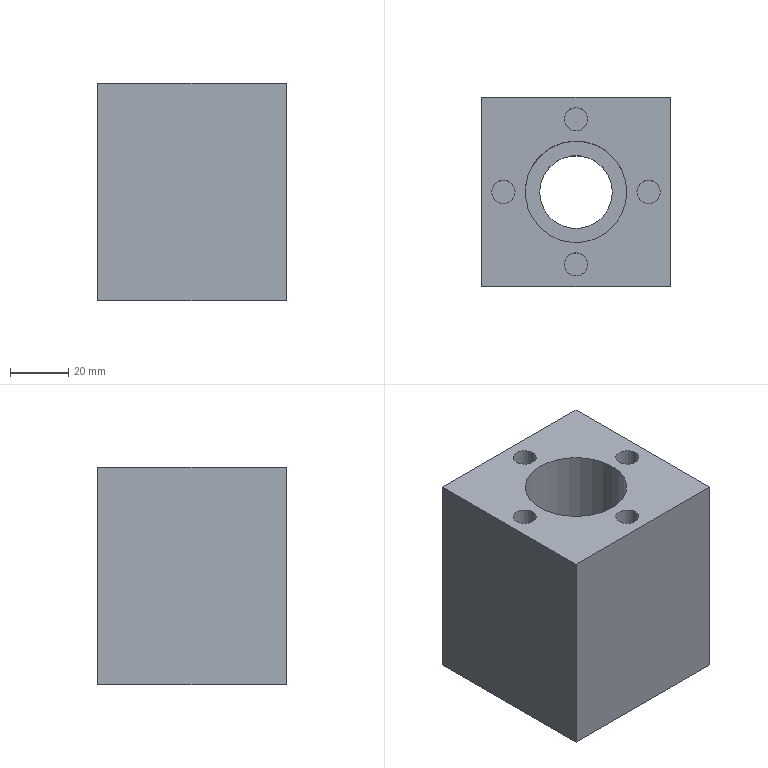Component | NX | BLANKDIEF | 1 solid | 17 faces | box 65 x 65 x 75 mm | volume 251446 mm3 | plane 11 | cylinder 6 | commonest cylinder face diameters 8 x4 25.025 x1 35 x1
STEP:
#1=CARTESIAN_POINT('',(0.,0.,0.));
#2=DIRECTION('',(0.,0.,1.));
#3=DIRECTION('',(1.,0.,0.));
#4=AXIS2_PLACEMENT_3D('',#1,#2,#3);
#5=CARTESIAN_POINT('',(-32.5,-105.5,73.077));
#6=VERTEX_POINT('',#5);
#7=CARTESIAN_POINT('',(32.5,-105.5,73.077));
#8=VERTEX_POINT('',#7);
#9=CARTESIAN_POINT('',(-32.5,-105.5,73.077));
#10=DIRECTION('',(1.,0.,0.));
#11=VECTOR('',#10,1.);
#12=LINE('',#9,#11);
#13=CARTESIAN_POINT('',(-32.5,-105.5,98.077));
#14=DIRECTION('',(-0.,1.,0.));
#15=DIRECTION('',(-1.,-0.,0.));
#16=AXIS2_PLACEMENT_3D('',#13,#14,#15);
#17=PLANE('',#16);
#18=CARTESIAN_POINT('',(0.,-25.));
#19=DIRECTION('',(-1.,0.));
#20=VECTOR('',#19,1.);
#21=LINE('',#18,#20);
#22=(GEOMETRIC_REPRESENTATION_CONTEXT(2)PARAMETRIC_REPRESENTATION_CONTEXT()REPRESENTATION_CONTEXT('',''));
#23=DEFINITIONAL_REPRESENTATION('',(#21),#22);
#24=PCURVE('',#17,#23);
#25=CARTESIAN_POINT('',(-0.,-73.,73.077));
#26=DIRECTION('',(0.,0.,-1.));
#27=DIRECTION('',(-1.,0.,0.));
#28=AXIS2_PLACEMENT_3D('',#25,#26,#27);
#29=PLANE('',#28);
#30=CARTESIAN_POINT('',(32.5,-32.5));
#31=DIRECTION('',(-1.,0.));
#32=VECTOR('',#31,1.);
#33=LINE('',#30,#32);
#34=(GEOMETRIC_REPRESENTATION_CONTEXT(2)PARAMETRIC_REPRESENTATION_CONTEXT()REPRESENTATION_CONTEXT('',''));
#35=DEFINITIONAL_REPRESENTATION('',(#33),#34);
#36=PCURVE('',#29,#35);
#37=SURFACE_CURVE('',#12,(#24,#36),.PCURVE_S1.);
#38=EDGE_CURVE('',#6,#8,#37,.T.);
#39=ORIENTED_EDGE('',*,*,#38,.T.);
#40=CARTESIAN_POINT('',(32.5,-105.5,148.077));
#41=VERTEX_POINT('',#40);
#42=CARTESIAN_POINT('',(32.5,-105.5,98.077));
#43=DIRECTION('',(0.,0.,-1.));
#44=VECTOR('',#43,1.);
#45=LINE('',#42,#44);
#46=CARTESIAN_POINT('',(-65.,0.));
#47=DIRECTION('',(0.,-1.));
#48=VECTOR('',#47,1.);
#49=LINE('',#46,#48);
#50=(GEOMETRIC_REPRESENTATION_CONTEXT(2)PARAMETRIC_REPRESENTATION_CONTEXT()REPRESENTATION_CONTEXT('',''));
#51=DEFINITIONAL_REPRESENTATION('',(#49),#50);
#52=PCURVE('',#17,#51);
#53=CARTESIAN_POINT('',(32.5,-105.5,98.077));
#54=DIRECTION('',(-1.,-0.,0.));
#55=DIRECTION('',(0.,-1.,0.));
#56=AXIS2_PLACEMENT_3D('',#53,#54,#55);
#57=PLANE('',#56);
#58=CARTESIAN_POINT('',(0.,0.));
#59=DIRECTION('',(0.,-1.));
#60=VECTOR('',#59,1.);
#61=LINE('',#58,#60);
#62=(GEOMETRIC_REPRESENTATION_CONTEXT(2)PARAMETRIC_REPRESENTATION_CONTEXT()REPRESENTATION_CONTEXT('',''));
#63=DEFINITIONAL_REPRESENTATION('',(#61),#62);
#64=PCURVE('',#57,#63);
#65=SURFACE_CURVE('',#45,(#52,#64),.PCURVE_S1.);
#66=EDGE_CURVE('',#41,#8,#65,.T.);
#67=ORIENTED_EDGE('',*,*,#66,.F.);
#68=CARTESIAN_POINT('',(-32.5,-105.5,148.077));
#69=VERTEX_POINT('',#68);
#70=CARTESIAN_POINT('',(32.5,-105.5,148.077));
#71=DIRECTION('',(-1.,0.,0.));
#72=VECTOR('',#71,1.);
#73=LINE('',#70,#72);
#74=CARTESIAN_POINT('',(-65.,50.));
#75=DIRECTION('',(1.,0.));
#76=VECTOR('',#75,1.);
#77=LINE('',#74,#76);
#78=(GEOMETRIC_REPRESENTATION_CONTEXT(2)PARAMETRIC_REPRESENTATION_CONTEXT()REPRESENTATION_CONTEXT('',''));
#79=DEFINITIONAL_REPRESENTATION('',(#77),#78);
#80=PCURVE('',#17,#79);
#81=CARTESIAN_POINT('',(-0.,-73.,148.077));
#82=DIRECTION('',(0.,0.,1.));
#83=DIRECTION('',(1.,0.,0.));
#84=AXIS2_PLACEMENT_3D('',#81,#82,#83);
#85=PLANE('',#84);
#86=CARTESIAN_POINT('',(32.5,-32.5));
#87=DIRECTION('',(-1.,0.));
#88=VECTOR('',#87,1.);
#89=LINE('',#86,#88);
#90=(GEOMETRIC_REPRESENTATION_CONTEXT(2)PARAMETRIC_REPRESENTATION_CONTEXT()REPRESENTATION_CONTEXT('',''));
#91=DEFINITIONAL_REPRESENTATION('',(#89),#90);
#92=PCURVE('',#85,#91);
#93=SURFACE_CURVE('',#73,(#80,#92),.PCURVE_S1.);
#94=EDGE_CURVE('',#41,#69,#93,.T.);
#95=ORIENTED_EDGE('',*,*,#94,.T.);
#96=CARTESIAN_POINT('',(-32.5,-105.5,98.077));
#97=DIRECTION('',(0.,0.,-1.));
#98=VECTOR('',#97,1.);
#99=LINE('',#96,#98);
#100=CARTESIAN_POINT('',(0.,0.));
#101=DIRECTION('',(0.,-1.));
#102=VECTOR('',#101,1.);
#103=LINE('',#100,#102);
#104=(GEOMETRIC_REPRESENTATION_CONTEXT(2)PARAMETRIC_REPRESENTATION_CONTEXT()REPRESENTATION_CONTEXT('',''));
#105=DEFINITIONAL_REPRESENTATION('',(#103),#104);
#106=PCURVE('',#17,#105);
#107=CARTESIAN_POINT('',(-32.5,-40.5,98.077));
#108=DIRECTION('',(1.,0.,0.));
#109=DIRECTION('',(-0.,1.,0.));
#110=AXIS2_PLACEMENT_3D('',#107,#108,#109);
#111=PLANE('',#110);
#112=CARTESIAN_POINT('',(-65.,0.));
#113=DIRECTION('',(0.,-1.));
#114=VECTOR('',#113,1.);
#115=LINE('',#112,#114);
#116=(GEOMETRIC_REPRESENTATION_CONTEXT(2)PARAMETRIC_REPRESENTATION_CONTEXT()REPRESENTATION_CONTEXT('',''));
#117=DEFINITIONAL_REPRESENTATION('',(#115),#116);
#118=PCURVE('',#111,#117);
#119=SURFACE_CURVE('',#99,(#106,#118),.PCURVE_S1.);
#120=EDGE_CURVE('',#69,#6,#119,.T.);
#121=ORIENTED_EDGE('',*,*,#120,.T.);
#122=EDGE_LOOP('',(#39,#67,#95,#121));
#123=FACE_BOUND('',#122,.T.);
#124=ADVANCED_FACE('',(#123),#17,.F.);
#125=CARTESIAN_POINT('',(32.5,-40.5,73.077));
#126=VERTEX_POINT('',#125);
#127=CARTESIAN_POINT('',(32.5,-105.5,73.077));
#128=DIRECTION('',(-0.,1.,0.));
#129=VECTOR('',#128,1.);
#130=LINE('',#127,#129);
#131=CARTESIAN_POINT('',(0.,-25.));
#132=DIRECTION('',(-1.,0.));
#133=VECTOR('',#132,1.);
#134=LINE('',#131,#133);
#135=(GEOMETRIC_REPRESENTATION_CONTEXT(2)PARAMETRIC_REPRESENTATION_CONTEXT()REPRESENTATION_CONTEXT('',''));
#136=DEFINITIONAL_REPRESENTATION('',(#134),#135);
#137=PCURVE('',#57,#136);
#138=CARTESIAN_POINT('',(-32.5,-32.5));
#139=DIRECTION('',(0.,1.));
#140=VECTOR('',#139,1.);
#141=LINE('',#138,#140);
#142=(GEOMETRIC_REPRESENTATION_CONTEXT(2)PARAMETRIC_REPRESENTATION_CONTEXT()REPRESENTATION_CONTEXT('',''));
#143=DEFINITIONAL_REPRESENTATION('',(#141),#142);
#144=PCURVE('',#29,#143);
#145=SURFACE_CURVE('',#130,(#137,#144),.PCURVE_S1.);
#146=EDGE_CURVE('',#8,#126,#145,.T.);
#147=ORIENTED_EDGE('',*,*,#146,.T.);
#148=CARTESIAN_POINT('',(32.5,-40.5,148.077));
#149=VERTEX_POINT('',#148);
#150=CARTESIAN_POINT('',(32.5,-40.5,98.077));
#151=DIRECTION('',(0.,0.,-1.));
#152=VECTOR('',#151,1.);
#153=LINE('',#150,#152);
#154=CARTESIAN_POINT('',(-65.,0.));
#155=DIRECTION('',(0.,-1.));
#156=VECTOR('',#155,1.);
#157=LINE('',#154,#156);
#158=(GEOMETRIC_REPRESENTATION_CONTEXT(2)PARAMETRIC_REPRESENTATION_CONTEXT()REPRESENTATION_CONTEXT('',''));
#159=DEFINITIONAL_REPRESENTATION('',(#157),#158);
#160=PCURVE('',#57,#159);
#161=CARTESIAN_POINT('',(32.5,-40.5,98.077));
#162=DIRECTION('',(0.,-1.,0.));
#163=DIRECTION('',(1.,0.,0.));
#164=AXIS2_PLACEMENT_3D('',#161,#162,#163);
#165=PLANE('',#164);
#166=CARTESIAN_POINT('',(0.,0.));
#167=DIRECTION('',(0.,-1.));
#168=VECTOR('',#167,1.);
#169=LINE('',#166,#168);
#170=(GEOMETRIC_REPRESENTATION_CONTEXT(2)PARAMETRIC_REPRESENTATION_CONTEXT()REPRESENTATION_CONTEXT('',''));
#171=DEFINITIONAL_REPRESENTATION('',(#169),#170);
#172=PCURVE('',#165,#171);
#173=SURFACE_CURVE('',#153,(#160,#172),.PCURVE_S1.);
#174=EDGE_CURVE('',#149,#126,#173,.T.);
#175=ORIENTED_EDGE('',*,*,#174,.F.);
#176=CARTESIAN_POINT('',(32.5,-40.5,148.077));
#177=DIRECTION('',(-0.,-1.,0.));
#178=VECTOR('',#177,1.);
#179=LINE('',#176,#178);
#180=CARTESIAN_POINT('',(-65.,50.));
#181=DIRECTION('',(1.,0.));
#182=VECTOR('',#181,1.);
#183=LINE('',#180,#182);
#184=(GEOMETRIC_REPRESENTATION_CONTEXT(2)PARAMETRIC_REPRESENTATION_CONTEXT()REPRESENTATION_CONTEXT('',''));
#185=DEFINITIONAL_REPRESENTATION('',(#183),#184);
#186=PCURVE('',#57,#185);
#187=CARTESIAN_POINT('',(32.5,32.5));
#188=DIRECTION('',(-0.,-1.));
#189=VECTOR('',#188,1.);
#190=LINE('',#187,#189);
#191=(GEOMETRIC_REPRESENTATION_CONTEXT(2)PARAMETRIC_REPRESENTATION_CONTEXT()REPRESENTATION_CONTEXT('',''));
#192=DEFINITIONAL_REPRESENTATION('',(#190),#191);
#193=PCURVE('',#85,#192);
#194=SURFACE_CURVE('',#179,(#186,#193),.PCURVE_S1.);
#195=EDGE_CURVE('',#149,#41,#194,.T.);
#196=ORIENTED_EDGE('',*,*,#195,.T.);
#197=ORIENTED_EDGE('',*,*,#66,.T.);
#198=EDGE_LOOP('',(#147,#175,#196,#197));
#199=FACE_BOUND('',#198,.T.);
#200=ADVANCED_FACE('',(#199),#57,.F.);
#201=CARTESIAN_POINT('',(-32.5,-40.5,73.077));
#202=VERTEX_POINT('',#201);
#203=CARTESIAN_POINT('',(32.5,-40.5,73.077));
#204=DIRECTION('',(-1.,-0.,0.));
#205=VECTOR('',#204,1.);
#206=LINE('',#203,#205);
#207=CARTESIAN_POINT('',(0.,-25.));
#208=DIRECTION('',(-1.,0.));
#209=VECTOR('',#208,1.);
#210=LINE('',#207,#209);
#211=(GEOMETRIC_REPRESENTATION_CONTEXT(2)PARAMETRIC_REPRESENTATION_CONTEXT()REPRESENTATION_CONTEXT('',''));
#212=DEFINITIONAL_REPRESENTATION('',(#210),#211);
#213=PCURVE('',#165,#212);
#214=CARTESIAN_POINT('',(-32.5,32.5));
#215=DIRECTION('',(1.,-0.));
#216=VECTOR('',#215,1.);
#217=LINE('',#214,#216);
#218=(GEOMETRIC_REPRESENTATION_CONTEXT(2)PARAMETRIC_REPRESENTATION_CONTEXT()REPRESENTATION_CONTEXT('',''));
#219=DEFINITIONAL_REPRESENTATION('',(#217),#218);
#220=PCURVE('',#29,#219);
#221=SURFACE_CURVE('',#206,(#213,#220),.PCURVE_S1.);
#222=EDGE_CURVE('',#126,#202,#221,.T.);
#223=ORIENTED_EDGE('',*,*,#222,.T.);
#224=CARTESIAN_POINT('',(-32.5,-40.5,148.077));
#225=VERTEX_POINT('',#224);
#226=CARTESIAN_POINT('',(-32.5,-40.5,98.077));
#227=DIRECTION('',(0.,0.,-1.));
#228=VECTOR('',#227,1.);
#229=LINE('',#226,#228);
#230=CARTESIAN_POINT('',(-65.,0.));
#231=DIRECTION('',(0.,-1.));
#232=VECTOR('',#231,1.);
#233=LINE('',#230,#232);
#234=(GEOMETRIC_REPRESENTATION_CONTEXT(2)PARAMETRIC_REPRESENTATION_CONTEXT()REPRESENTATION_CONTEXT('',''));
#235=DEFINITIONAL_REPRESENTATION('',(#233),#234);
#236=PCURVE('',#165,#235);
#237=CARTESIAN_POINT('',(0.,0.));
#238=DIRECTION('',(0.,-1.));
#239=VECTOR('',#238,1.);
#240=LINE('',#237,#239);
#241=(GEOMETRIC_REPRESENTATION_CONTEXT(2)PARAMETRIC_REPRESENTATION_CONTEXT()REPRESENTATION_CONTEXT('',''));
#242=DEFINITIONAL_REPRESENTATION('',(#240),#241);
#243=PCURVE('',#111,#242);
#244=SURFACE_CURVE('',#229,(#236,#243),.PCURVE_S1.);
#245=EDGE_CURVE('',#225,#202,#244,.T.);
#246=ORIENTED_EDGE('',*,*,#245,.F.);
#247=CARTESIAN_POINT('',(-32.5,-40.5,148.077));
#248=DIRECTION('',(1.,-0.,0.));
#249=VECTOR('',#248,1.);
#250=LINE('',#247,#249);
#251=CARTESIAN_POINT('',(-65.,50.));
#252=DIRECTION('',(1.,0.));
#253=VECTOR('',#252,1.);
#254=LINE('',#251,#253);
#255=(GEOMETRIC_REPRESENTATION_CONTEXT(2)PARAMETRIC_REPRESENTATION_CONTEXT()REPRESENTATION_CONTEXT('',''));
#256=DEFINITIONAL_REPRESENTATION('',(#254),#255);
#257=PCURVE('',#165,#256);
#258=CARTESIAN_POINT('',(-32.5,32.5));
#259=DIRECTION('',(1.,-0.));
#260=VECTOR('',#259,1.);
#261=LINE('',#258,#260);
#262=(GEOMETRIC_REPRESENTATION_CONTEXT(2)PARAMETRIC_REPRESENTATION_CONTEXT()REPRESENTATION_CONTEXT('',''));
#263=DEFINITIONAL_REPRESENTATION('',(#261),#262);
#264=PCURVE('',#85,#263);
#265=SURFACE_CURVE('',#250,(#257,#264),.PCURVE_S1.);
#266=EDGE_CURVE('',#225,#149,#265,.T.);
#267=ORIENTED_EDGE('',*,*,#266,.T.);
#268=ORIENTED_EDGE('',*,*,#174,.T.);
#269=EDGE_LOOP('',(#223,#246,#267,#268));
#270=FACE_BOUND('',#269,.T.);
#271=ADVANCED_FACE('',(#270),#165,.F.);
#272=CARTESIAN_POINT('',(-32.5,-40.5,73.077));
#273=DIRECTION('',(0.,-1.,0.));
#274=VECTOR('',#273,1.);
#275=LINE('',#272,#274);
#276=CARTESIAN_POINT('',(0.,-25.));
#277=DIRECTION('',(-1.,0.));
#278=VECTOR('',#277,1.);
#279=LINE('',#276,#278);
#280=(GEOMETRIC_REPRESENTATION_CONTEXT(2)PARAMETRIC_REPRESENTATION_CONTEXT()REPRESENTATION_CONTEXT('',''));
#281=DEFINITIONAL_REPRESENTATION('',(#279),#280);
#282=PCURVE('',#111,#281);
#283=CARTESIAN_POINT('',(32.5,32.5));
#284=DIRECTION('',(-0.,-1.));
#285=VECTOR('',#284,1.);
#286=LINE('',#283,#285);
#287=(GEOMETRIC_REPRESENTATION_CONTEXT(2)PARAMETRIC_REPRESENTATION_CONTEXT()REPRESENTATION_CONTEXT('',''));
#288=DEFINITIONAL_REPRESENTATION('',(#286),#287);
#289=PCURVE('',#29,#288);
#290=SURFACE_CURVE('',#275,(#282,#289),.PCURVE_S1.);
#291=EDGE_CURVE('',#202,#6,#290,.T.);
#292=ORIENTED_EDGE('',*,*,#291,.T.);
#293=ORIENTED_EDGE('',*,*,#120,.F.);
#294=CARTESIAN_POINT('',(-32.5,-105.5,148.077));
#295=DIRECTION('',(0.,1.,0.));
#296=VECTOR('',#295,1.);
#297=LINE('',#294,#296);
#298=CARTESIAN_POINT('',(-65.,50.));
#299=DIRECTION('',(1.,0.));
#300=VECTOR('',#299,1.);
#301=LINE('',#298,#300);
#302=(GEOMETRIC_REPRESENTATION_CONTEXT(2)PARAMETRIC_REPRESENTATION_CONTEXT()REPRESENTATION_CONTEXT('',''));
#303=DEFINITIONAL_REPRESENTATION('',(#301),#302);
#304=PCURVE('',#111,#303);
#305=CARTESIAN_POINT('',(-32.5,-32.5));
#306=DIRECTION('',(0.,1.));
#307=VECTOR('',#306,1.);
#308=LINE('',#305,#307);
#309=(GEOMETRIC_REPRESENTATION_CONTEXT(2)PARAMETRIC_REPRESENTATION_CONTEXT()REPRESENTATION_CONTEXT('',''));
#310=DEFINITIONAL_REPRESENTATION('',(#308),#309);
#311=PCURVE('',#85,#310);
#312=SURFACE_CURVE('',#297,(#304,#311),.PCURVE_S1.);
#313=EDGE_CURVE('',#69,#225,#312,.T.);
#314=ORIENTED_EDGE('',*,*,#313,.T.);
#315=ORIENTED_EDGE('',*,*,#245,.T.);
#316=EDGE_LOOP('',(#292,#293,#314,#315));
#317=FACE_BOUND('',#316,.T.);
#318=ADVANCED_FACE('',(#317),#111,.F.);
#319=CARTESIAN_POINT('',(12.512,-73.,98.077));
#320=VERTEX_POINT('',#319);
#321=CARTESIAN_POINT('',(-0.,-73.,98.077));
#322=DIRECTION('',(0.,0.,-1.));
#323=DIRECTION('',(1.,0.,0.));
#324=AXIS2_PLACEMENT_3D('',#321,#322,#323);
#325=CIRCLE('',#324,12.512);
#326=CARTESIAN_POINT('',(-0.,-73.,98.077));
#327=DIRECTION('',(0.,0.,-1.));
#328=DIRECTION('',(-1.,0.,0.));
#329=AXIS2_PLACEMENT_3D('',#326,#327,#328);
#330=CYLINDRICAL_SURFACE('',#329,12.512);
#331=CARTESIAN_POINT('',(3.142,0.));
#332=DIRECTION('',(1.,0.));
#333=VECTOR('',#332,1.);
#334=LINE('',#331,#333);
#335=(GEOMETRIC_REPRESENTATION_CONTEXT(2)PARAMETRIC_REPRESENTATION_CONTEXT()REPRESENTATION_CONTEXT('',''));
#336=DEFINITIONAL_REPRESENTATION('',(#334),#335);
#337=PCURVE('',#330,#336);
#338=CARTESIAN_POINT('',(-0.,-73.,98.077));
#339=DIRECTION('',(0.,0.,-1.));
#340=DIRECTION('',(-1.,0.,0.));
#341=AXIS2_PLACEMENT_3D('',#338,#339,#340);
#342=PLANE('',#341);
#343=CARTESIAN_POINT('',(0.,0.));
#344=DIRECTION('',(-1.,0.));
#345=AXIS2_PLACEMENT_2D('',#343,#344);
#346=CIRCLE('',#345,12.512);
#347=(GEOMETRIC_REPRESENTATION_CONTEXT(2)PARAMETRIC_REPRESENTATION_CONTEXT()REPRESENTATION_CONTEXT('',''));
#348=DEFINITIONAL_REPRESENTATION('',(#346),#347);
#349=PCURVE('',#342,#348);
#350=SURFACE_CURVE('',#325,(#337,#349),.PCURVE_S1.);
#351=EDGE_CURVE('',#320,#320,#350,.T.);
#352=ORIENTED_EDGE('',*,*,#351,.T.);
#353=CARTESIAN_POINT('',(12.512,-73.,73.077));
#354=VERTEX_POINT('',#353);
#355=CARTESIAN_POINT('',(12.512,-73.,98.077));
#356=CARTESIAN_POINT('',(12.512,-73.,73.077));
#357=B_SPLINE_CURVE_WITH_KNOTS('',1,(#355,#356),.UNSPECIFIED.,.F.,.F.,(2,2),(0.,25.),.PIECEWISE_BEZIER_KNOTS.);
#358=CARTESIAN_POINT('',(9.425,0.));
#359=DIRECTION('',(0.,1.));
#360=VECTOR('',#359,1.);
#361=LINE('',#358,#360);
#362=(GEOMETRIC_REPRESENTATION_CONTEXT(2)PARAMETRIC_REPRESENTATION_CONTEXT()REPRESENTATION_CONTEXT('',''));
#363=DEFINITIONAL_REPRESENTATION('',(#361),#362);
#364=PCURVE('',#330,#363);
#365=CARTESIAN_POINT('',(3.142,0.));
#366=DIRECTION('',(0.,1.));
#367=VECTOR('',#366,1.);
#368=LINE('',#365,#367);
#369=(GEOMETRIC_REPRESENTATION_CONTEXT(2)PARAMETRIC_REPRESENTATION_CONTEXT()REPRESENTATION_CONTEXT('',''));
#370=DEFINITIONAL_REPRESENTATION('',(#368),#369);
#371=PCURVE('',#330,#370);
#372=SEAM_CURVE('',#357,(#364,#371),.PCURVE_S1.);
#373=EDGE_CURVE('',#320,#354,#372,.T.);
#374=ORIENTED_EDGE('',*,*,#373,.T.);
#375=CARTESIAN_POINT('',(-0.,-73.,73.077));
#376=DIRECTION('',(0.,0.,-1.));
#377=DIRECTION('',(1.,0.,0.));
#378=AXIS2_PLACEMENT_3D('',#375,#376,#377);
#379=CIRCLE('',#378,12.512);
#380=CARTESIAN_POINT('',(3.142,25.));
#381=DIRECTION('',(1.,0.));
#382=VECTOR('',#381,1.);
#383=LINE('',#380,#382);
#384=(GEOMETRIC_REPRESENTATION_CONTEXT(2)PARAMETRIC_REPRESENTATION_CONTEXT()REPRESENTATION_CONTEXT('',''));
#385=DEFINITIONAL_REPRESENTATION('',(#383),#384);
#386=PCURVE('',#330,#385);
#387=CARTESIAN_POINT('',(0.,0.));
#388=DIRECTION('',(-1.,0.));
#389=AXIS2_PLACEMENT_2D('',#387,#388);
#390=CIRCLE('',#389,12.512);
#391=(GEOMETRIC_REPRESENTATION_CONTEXT(2)PARAMETRIC_REPRESENTATION_CONTEXT()REPRESENTATION_CONTEXT('',''));
#392=DEFINITIONAL_REPRESENTATION('',(#390),#391);
#393=PCURVE('',#29,#392);
#394=SURFACE_CURVE('',#379,(#386,#393),.PCURVE_S1.);
#395=EDGE_CURVE('',#354,#354,#394,.T.);
#396=ORIENTED_EDGE('',*,*,#395,.F.);
#397=ORIENTED_EDGE('',*,*,#373,.F.);
#398=EDGE_LOOP('',(#352,#374,#396,#397));
#399=FACE_BOUND('',#398,.F.);
#400=ADVANCED_FACE('',(#399),#330,.F.);
#401=CARTESIAN_POINT('',(17.5,-73.,98.077));
#402=VERTEX_POINT('',#401);
#403=CARTESIAN_POINT('',(-0.,-73.,98.077));
#404=DIRECTION('',(0.,0.,1.));
#405=DIRECTION('',(1.,0.,0.));
#406=AXIS2_PLACEMENT_3D('',#403,#404,#405);
#407=CIRCLE('',#406,17.5);
#408=CARTESIAN_POINT('',(-17.5,0.));
#409=CARTESIAN_POINT('',(-17.5,30.311));
#410=CARTESIAN_POINT('',(8.75,15.155));
#411=CARTESIAN_POINT('',(35.,0.));
#412=CARTESIAN_POINT('',(8.75,-15.155));
#413=CARTESIAN_POINT('',(-17.5,-30.311));
#414=CARTESIAN_POINT('',(-17.5,0.));
#415=(BOUNDED_CURVE()B_SPLINE_CURVE(2,(#408,#409,#410,#411,#412,#413,#414),.UNSPECIFIED.,.T.,.F.)B_SPLINE_CURVE_WITH_KNOTS((1,2,2,2,2,1),(-2.094,0.,2.094,4.189,6.283,8.378),.UNSPECIFIED.)CURVE()GEOMETRIC_REPRESENTATION_ITEM()RATIONAL_B_SPLINE_CURVE((1.,0.5,1.,0.5,1.,0.5,1.))REPRESENTATION_ITEM(''));
#416=(GEOMETRIC_REPRESENTATION_CONTEXT(2)PARAMETRIC_REPRESENTATION_CONTEXT()REPRESENTATION_CONTEXT('',''));
#417=DEFINITIONAL_REPRESENTATION('',(#415),#416);
#418=PCURVE('',#342,#417);
#419=CARTESIAN_POINT('',(-0.,-73.,148.077));
#420=DIRECTION('',(0.,0.,-1.));
#421=DIRECTION('',(-1.,0.,0.));
#422=AXIS2_PLACEMENT_3D('',#419,#420,#421);
#423=CYLINDRICAL_SURFACE('',#422,17.5);
#424=CARTESIAN_POINT('',(9.425,50.));
#425=DIRECTION('',(-1.,0.));
#426=VECTOR('',#425,1.);
#427=LINE('',#424,#426);
#428=(GEOMETRIC_REPRESENTATION_CONTEXT(2)PARAMETRIC_REPRESENTATION_CONTEXT()REPRESENTATION_CONTEXT('',''));
#429=DEFINITIONAL_REPRESENTATION('',(#427),#428);
#430=PCURVE('',#423,#429);
#431=SURFACE_CURVE('',#407,(#418,#430),.PCURVE_S1.);
#432=EDGE_CURVE('',#402,#402,#431,.T.);
#433=ORIENTED_EDGE('',*,*,#432,.T.);
#434=EDGE_LOOP('',(#433));
#435=FACE_BOUND('',#434,.T.);
#436=ORIENTED_EDGE('',*,*,#351,.T.);
#437=EDGE_LOOP('',(#436));
#438=FACE_BOUND('',#437,.T.);
#439=ADVANCED_FACE('',(#435,#438),#342,.F.);
#440=ORIENTED_EDGE('',*,*,#38,.F.);
#441=ORIENTED_EDGE('',*,*,#291,.F.);
#442=ORIENTED_EDGE('',*,*,#222,.F.);
#443=ORIENTED_EDGE('',*,*,#146,.F.);
#444=EDGE_LOOP('',(#440,#441,#442,#443));
#445=FACE_BOUND('',#444,.T.);
#446=ORIENTED_EDGE('',*,*,#395,.F.);
#447=EDGE_LOOP('',(#446));
#448=FACE_BOUND('',#447,.T.);
#449=ADVANCED_FACE('',(#445,#448),#29,.T.);
#450=CARTESIAN_POINT('',(17.5,-73.,148.077));
#451=VERTEX_POINT('',#450);
#452=CARTESIAN_POINT('',(-0.,-73.,148.077));
#453=DIRECTION('',(0.,0.,1.));
#454=DIRECTION('',(1.,0.,0.));
#455=AXIS2_PLACEMENT_3D('',#452,#453,#454);
#456=CIRCLE('',#455,17.5);
#457=CARTESIAN_POINT('',(9.425,0.));
#458=DIRECTION('',(-1.,0.));
#459=VECTOR('',#458,1.);
#460=LINE('',#457,#459);
#461=(GEOMETRIC_REPRESENTATION_CONTEXT(2)PARAMETRIC_REPRESENTATION_CONTEXT()REPRESENTATION_CONTEXT('',''));
#462=DEFINITIONAL_REPRESENTATION('',(#460),#461);
#463=PCURVE('',#423,#462);
#464=CARTESIAN_POINT('',(0.,0.));
#465=DIRECTION('',(1.,0.));
#466=AXIS2_PLACEMENT_2D('',#464,#465);
#467=CIRCLE('',#466,17.5);
#468=(GEOMETRIC_REPRESENTATION_CONTEXT(2)PARAMETRIC_REPRESENTATION_CONTEXT()REPRESENTATION_CONTEXT('',''));
#469=DEFINITIONAL_REPRESENTATION('',(#467),#468);
#470=PCURVE('',#85,#469);
#471=SURFACE_CURVE('',#456,(#463,#470),.PCURVE_S1.);
#472=EDGE_CURVE('',#451,#451,#471,.T.);
#473=ORIENTED_EDGE('',*,*,#472,.F.);
#474=CARTESIAN_POINT('',(17.5,-73.,148.077));
#475=CARTESIAN_POINT('',(17.5,-73.,98.077));
#476=B_SPLINE_CURVE_WITH_KNOTS('',1,(#474,#475),.UNSPECIFIED.,.F.,.F.,(2,2),(0.,50.),.PIECEWISE_BEZIER_KNOTS.);
#477=CARTESIAN_POINT('',(9.425,0.));
#478=DIRECTION('',(0.,1.));
#479=VECTOR('',#478,1.);
#480=LINE('',#477,#479);
#481=(GEOMETRIC_REPRESENTATION_CONTEXT(2)PARAMETRIC_REPRESENTATION_CONTEXT()REPRESENTATION_CONTEXT('',''));
#482=DEFINITIONAL_REPRESENTATION('',(#480),#481);
#483=PCURVE('',#423,#482);
#484=CARTESIAN_POINT('',(3.142,0.));
#485=DIRECTION('',(0.,1.));
#486=VECTOR('',#485,1.);
#487=LINE('',#484,#486);
#488=(GEOMETRIC_REPRESENTATION_CONTEXT(2)PARAMETRIC_REPRESENTATION_CONTEXT()REPRESENTATION_CONTEXT('',''));
#489=DEFINITIONAL_REPRESENTATION('',(#487),#488);
#490=PCURVE('',#423,#489);
#491=SEAM_CURVE('',#476,(#483,#490),.PCURVE_S1.);
#492=EDGE_CURVE('',#451,#402,#491,.T.);
#493=ORIENTED_EDGE('',*,*,#492,.T.);
#494=ORIENTED_EDGE('',*,*,#432,.T.);
#495=ORIENTED_EDGE('',*,*,#492,.F.);
#496=EDGE_LOOP('',(#473,#493,#494,#495));
#497=FACE_BOUND('',#496,.F.);
#498=ADVANCED_FACE('',(#497),#423,.F.);
#499=CARTESIAN_POINT('',(-21.,-73.,148.077));
#500=VERTEX_POINT('',#499);
#501=CARTESIAN_POINT('',(-25.,-73.,148.077));
#502=DIRECTION('',(0.,0.,1.));
#503=DIRECTION('',(1.,0.,0.));
#504=AXIS2_PLACEMENT_3D('',#501,#502,#503);
#505=CIRCLE('',#504,4.);
#506=CARTESIAN_POINT('',(-25.,0.));
#507=DIRECTION('',(1.,0.));
#508=AXIS2_PLACEMENT_2D('',#506,#507);
#509=CIRCLE('',#508,4.);
#510=(GEOMETRIC_REPRESENTATION_CONTEXT(2)PARAMETRIC_REPRESENTATION_CONTEXT()REPRESENTATION_CONTEXT('',''));
#511=DEFINITIONAL_REPRESENTATION('',(#509),#510);
#512=PCURVE('',#85,#511);
#513=CARTESIAN_POINT('',(-25.,-73.,123.077));
#514=DIRECTION('',(0.,0.,1.));
#515=DIRECTION('',(1.,0.,0.));
#516=AXIS2_PLACEMENT_3D('',#513,#514,#515);
#517=CYLINDRICAL_SURFACE('',#516,4.);
#518=CARTESIAN_POINT('',(0.,25.));
#519=DIRECTION('',(1.,0.));
#520=VECTOR('',#519,1.);
#521=LINE('',#518,#520);
#522=(GEOMETRIC_REPRESENTATION_CONTEXT(2)PARAMETRIC_REPRESENTATION_CONTEXT()REPRESENTATION_CONTEXT('',''));
#523=DEFINITIONAL_REPRESENTATION('',(#521),#522);
#524=PCURVE('',#517,#523);
#525=SURFACE_CURVE('',#505,(#512,#524),.PCURVE_S1.);
#526=EDGE_CURVE('',#500,#500,#525,.T.);
#527=ORIENTED_EDGE('',*,*,#526,.F.);
#528=EDGE_LOOP('',(#527));
#529=FACE_BOUND('',#528,.T.);
#530=CARTESIAN_POINT('',(4.,-98.,148.077));
#531=VERTEX_POINT('',#530);
#532=CARTESIAN_POINT('',(-0.,-98.,148.077));
#533=DIRECTION('',(0.,0.,1.));
#534=DIRECTION('',(1.,0.,0.));
#535=AXIS2_PLACEMENT_3D('',#532,#533,#534);
#536=CIRCLE('',#535,4.);
#537=CARTESIAN_POINT('',(0.,-25.));
#538=DIRECTION('',(1.,0.));
#539=AXIS2_PLACEMENT_2D('',#537,#538);
#540=CIRCLE('',#539,4.);
#541=(GEOMETRIC_REPRESENTATION_CONTEXT(2)PARAMETRIC_REPRESENTATION_CONTEXT()REPRESENTATION_CONTEXT('',''));
#542=DEFINITIONAL_REPRESENTATION('',(#540),#541);
#543=PCURVE('',#85,#542);
#544=CARTESIAN_POINT('',(-0.,-98.,123.077));
#545=DIRECTION('',(0.,0.,1.));
#546=DIRECTION('',(1.,0.,0.));
#547=AXIS2_PLACEMENT_3D('',#544,#545,#546);
#548=CYLINDRICAL_SURFACE('',#547,4.);
#549=CARTESIAN_POINT('',(0.,25.));
#550=DIRECTION('',(1.,0.));
#551=VECTOR('',#550,1.);
#552=LINE('',#549,#551);
#553=(GEOMETRIC_REPRESENTATION_CONTEXT(2)PARAMETRIC_REPRESENTATION_CONTEXT()REPRESENTATION_CONTEXT('',''));
#554=DEFINITIONAL_REPRESENTATION('',(#552),#553);
#555=PCURVE('',#548,#554);
#556=SURFACE_CURVE('',#536,(#543,#555),.PCURVE_S1.);
#557=EDGE_CURVE('',#531,#531,#556,.T.);
#558=ORIENTED_EDGE('',*,*,#557,.F.);
#559=EDGE_LOOP('',(#558));
#560=FACE_BOUND('',#559,.T.);
#561=CARTESIAN_POINT('',(4.,-48.,148.077));
#562=VERTEX_POINT('',#561);
#563=CARTESIAN_POINT('',(-0.,-48.,148.077));
#564=DIRECTION('',(0.,0.,1.));
#565=DIRECTION('',(1.,0.,0.));
#566=AXIS2_PLACEMENT_3D('',#563,#564,#565);
#567=CIRCLE('',#566,4.);
#568=CARTESIAN_POINT('',(0.,25.));
#569=DIRECTION('',(1.,0.));
#570=AXIS2_PLACEMENT_2D('',#568,#569);
#571=CIRCLE('',#570,4.);
#572=(GEOMETRIC_REPRESENTATION_CONTEXT(2)PARAMETRIC_REPRESENTATION_CONTEXT()REPRESENTATION_CONTEXT('',''));
#573=DEFINITIONAL_REPRESENTATION('',(#571),#572);
#574=PCURVE('',#85,#573);
#575=CARTESIAN_POINT('',(-0.,-48.,123.077));
#576=DIRECTION('',(0.,0.,1.));
#577=DIRECTION('',(1.,0.,0.));
#578=AXIS2_PLACEMENT_3D('',#575,#576,#577);
#579=CYLINDRICAL_SURFACE('',#578,4.);
#580=CARTESIAN_POINT('',(0.,25.));
#581=DIRECTION('',(1.,0.));
#582=VECTOR('',#581,1.);
#583=LINE('',#580,#582);
#584=(GEOMETRIC_REPRESENTATION_CONTEXT(2)PARAMETRIC_REPRESENTATION_CONTEXT()REPRESENTATION_CONTEXT('',''));
#585=DEFINITIONAL_REPRESENTATION('',(#583),#584);
#586=PCURVE('',#579,#585);
#587=SURFACE_CURVE('',#567,(#574,#586),.PCURVE_S1.);
#588=EDGE_CURVE('',#562,#562,#587,.T.);
#589=ORIENTED_EDGE('',*,*,#588,.F.);
#590=EDGE_LOOP('',(#589));
#591=FACE_BOUND('',#590,.T.);
#592=CARTESIAN_POINT('',(29.,-73.,148.077));
#593=VERTEX_POINT('',#592);
#594=CARTESIAN_POINT('',(25.,-73.,148.077));
#595=DIRECTION('',(0.,0.,1.));
#596=DIRECTION('',(1.,0.,0.));
#597=AXIS2_PLACEMENT_3D('',#594,#595,#596);
#598=CIRCLE('',#597,4.);
#599=CARTESIAN_POINT('',(25.,0.));
#600=DIRECTION('',(1.,0.));
#601=AXIS2_PLACEMENT_2D('',#599,#600);
#602=CIRCLE('',#601,4.);
#603=(GEOMETRIC_REPRESENTATION_CONTEXT(2)PARAMETRIC_REPRESENTATION_CONTEXT()REPRESENTATION_CONTEXT('',''));
#604=DEFINITIONAL_REPRESENTATION('',(#602),#603);
#605=PCURVE('',#85,#604);
#606=CARTESIAN_POINT('',(25.,-73.,123.077));
#607=DIRECTION('',(0.,0.,1.));
#608=DIRECTION('',(1.,0.,0.));
#609=AXIS2_PLACEMENT_3D('',#606,#607,#608);
#610=CYLINDRICAL_SURFACE('',#609,4.);
#611=CARTESIAN_POINT('',(0.,25.));
#612=DIRECTION('',(1.,0.));
#613=VECTOR('',#612,1.);
#614=LINE('',#611,#613);
#615=(GEOMETRIC_REPRESENTATION_CONTEXT(2)PARAMETRIC_REPRESENTATION_CONTEXT()REPRESENTATION_CONTEXT('',''));
#616=DEFINITIONAL_REPRESENTATION('',(#614),#615);
#617=PCURVE('',#610,#616);
#618=SURFACE_CURVE('',#598,(#605,#617),.PCURVE_S1.);
#619=EDGE_CURVE('',#593,#593,#618,.T.);
#620=ORIENTED_EDGE('',*,*,#619,.F.);
#621=EDGE_LOOP('',(#620));
#622=FACE_BOUND('',#621,.T.);
#623=ORIENTED_EDGE('',*,*,#313,.F.);
#624=ORIENTED_EDGE('',*,*,#94,.F.);
#625=ORIENTED_EDGE('',*,*,#195,.F.);
#626=ORIENTED_EDGE('',*,*,#266,.F.);
#627=EDGE_LOOP('',(#623,#624,#625,#626));
#628=FACE_BOUND('',#627,.T.);
#629=ORIENTED_EDGE('',*,*,#472,.F.);
#630=EDGE_LOOP('',(#629));
#631=FACE_BOUND('',#630,.T.);
#632=ADVANCED_FACE('',(#529,#560,#591,#622,#628,#631),#85,.T.);
#633=CARTESIAN_POINT('',(29.,-73.,123.077));
#634=VERTEX_POINT('',#633);
#635=CARTESIAN_POINT('',(25.,-73.,123.077));
#636=DIRECTION('',(0.,0.,-1.));
#637=DIRECTION('',(1.,0.,0.));
#638=AXIS2_PLACEMENT_3D('',#635,#636,#637);
#639=CIRCLE('',#638,4.);
#640=CARTESIAN_POINT('',(6.283,0.));
#641=DIRECTION('',(-1.,0.));
#642=VECTOR('',#641,1.);
#643=LINE('',#640,#642);
#644=(GEOMETRIC_REPRESENTATION_CONTEXT(2)PARAMETRIC_REPRESENTATION_CONTEXT()REPRESENTATION_CONTEXT('',''));
#645=DEFINITIONAL_REPRESENTATION('',(#643),#644);
#646=PCURVE('',#610,#645);
#647=CARTESIAN_POINT('',(25.,-73.,123.077));
#648=DIRECTION('',(0.,0.,1.));
#649=DIRECTION('',(1.,0.,0.));
#650=AXIS2_PLACEMENT_3D('',#647,#648,#649);
#651=PLANE('',#650);
#652=CARTESIAN_POINT('',(4.,0.));
#653=CARTESIAN_POINT('',(4.,-6.928));
#654=CARTESIAN_POINT('',(-2.,-3.464));
#655=CARTESIAN_POINT('',(-8.,-0.));
#656=CARTESIAN_POINT('',(-2.,3.464));
#657=CARTESIAN_POINT('',(4.,6.928));
#658=CARTESIAN_POINT('',(4.,0.));
#659=(BOUNDED_CURVE()B_SPLINE_CURVE(2,(#652,#653,#654,#655,#656,#657,#658),.UNSPECIFIED.,.T.,.F.)B_SPLINE_CURVE_WITH_KNOTS((1,2,2,2,2,1),(-2.094,0.,2.094,4.189,6.283,8.378),.UNSPECIFIED.)CURVE()GEOMETRIC_REPRESENTATION_ITEM()RATIONAL_B_SPLINE_CURVE((1.,0.5,1.,0.5,1.,0.5,1.))REPRESENTATION_ITEM(''));
#660=(GEOMETRIC_REPRESENTATION_CONTEXT(2)PARAMETRIC_REPRESENTATION_CONTEXT()REPRESENTATION_CONTEXT('',''));
#661=DEFINITIONAL_REPRESENTATION('',(#659),#660);
#662=PCURVE('',#651,#661);
#663=SURFACE_CURVE('',#639,(#646,#662),.PCURVE_S1.);
#664=EDGE_CURVE('',#634,#634,#663,.T.);
#665=ORIENTED_EDGE('',*,*,#664,.F.);
#666=CARTESIAN_POINT('',(29.,-73.,123.077));
#667=CARTESIAN_POINT('',(29.,-73.,148.077));
#668=B_SPLINE_CURVE_WITH_KNOTS('',1,(#666,#667),.UNSPECIFIED.,.F.,.F.,(2,2),(0.,25.),.PIECEWISE_BEZIER_KNOTS.);
#669=CARTESIAN_POINT('',(6.283,0.));
#670=DIRECTION('',(0.,1.));
#671=VECTOR('',#670,1.);
#672=LINE('',#669,#671);
#673=(GEOMETRIC_REPRESENTATION_CONTEXT(2)PARAMETRIC_REPRESENTATION_CONTEXT()REPRESENTATION_CONTEXT('',''));
#674=DEFINITIONAL_REPRESENTATION('',(#672),#673);
#675=PCURVE('',#610,#674);
#676=CARTESIAN_POINT('',(0.,0.));
#677=DIRECTION('',(0.,1.));
#678=VECTOR('',#677,1.);
#679=LINE('',#676,#678);
#680=(GEOMETRIC_REPRESENTATION_CONTEXT(2)PARAMETRIC_REPRESENTATION_CONTEXT()REPRESENTATION_CONTEXT('',''));
#681=DEFINITIONAL_REPRESENTATION('',(#679),#680);
#682=PCURVE('',#610,#681);
#683=SEAM_CURVE('',#668,(#675,#682),.PCURVE_S1.);
#684=EDGE_CURVE('',#634,#593,#683,.T.);
#685=ORIENTED_EDGE('',*,*,#684,.T.);
#686=ORIENTED_EDGE('',*,*,#619,.F.);
#687=ORIENTED_EDGE('',*,*,#684,.F.);
#688=EDGE_LOOP('',(#665,#685,#686,#687));
#689=FACE_BOUND('',#688,.F.);
#690=ADVANCED_FACE('',(#689),#610,.F.);
#691=ORIENTED_EDGE('',*,*,#664,.F.);
#692=EDGE_LOOP('',(#691));
#693=FACE_BOUND('',#692,.T.);
#694=ADVANCED_FACE('',(#693),#651,.T.);
#695=CARTESIAN_POINT('',(4.,-48.,123.077));
#696=VERTEX_POINT('',#695);
#697=CARTESIAN_POINT('',(-0.,-48.,123.077));
#698=DIRECTION('',(0.,0.,-1.));
#699=DIRECTION('',(1.,0.,0.));
#700=AXIS2_PLACEMENT_3D('',#697,#698,#699);
#701=CIRCLE('',#700,4.);
#702=CARTESIAN_POINT('',(6.283,0.));
#703=DIRECTION('',(-1.,0.));
#704=VECTOR('',#703,1.);
#705=LINE('',#702,#704);
#706=(GEOMETRIC_REPRESENTATION_CONTEXT(2)PARAMETRIC_REPRESENTATION_CONTEXT()REPRESENTATION_CONTEXT('',''));
#707=DEFINITIONAL_REPRESENTATION('',(#705),#706);
#708=PCURVE('',#579,#707);
#709=CARTESIAN_POINT('',(-0.,-48.,123.077));
#710=DIRECTION('',(0.,0.,1.));
#711=DIRECTION('',(1.,0.,0.));
#712=AXIS2_PLACEMENT_3D('',#709,#710,#711);
#713=PLANE('',#712);
#714=CARTESIAN_POINT('',(4.,0.));
#715=CARTESIAN_POINT('',(4.,-6.928));
#716=CARTESIAN_POINT('',(-2.,-3.464));
#717=CARTESIAN_POINT('',(-8.,-0.));
#718=CARTESIAN_POINT('',(-2.,3.464));
#719=CARTESIAN_POINT('',(4.,6.928));
#720=CARTESIAN_POINT('',(4.,0.));
#721=(BOUNDED_CURVE()B_SPLINE_CURVE(2,(#714,#715,#716,#717,#718,#719,#720),.UNSPECIFIED.,.T.,.F.)B_SPLINE_CURVE_WITH_KNOTS((1,2,2,2,2,1),(-2.094,0.,2.094,4.189,6.283,8.378),.UNSPECIFIED.)CURVE()GEOMETRIC_REPRESENTATION_ITEM()RATIONAL_B_SPLINE_CURVE((1.,0.5,1.,0.5,1.,0.5,1.))REPRESENTATION_ITEM(''));
#722=(GEOMETRIC_REPRESENTATION_CONTEXT(2)PARAMETRIC_REPRESENTATION_CONTEXT()REPRESENTATION_CONTEXT('',''));
#723=DEFINITIONAL_REPRESENTATION('',(#721),#722);
#724=PCURVE('',#713,#723);
#725=SURFACE_CURVE('',#701,(#708,#724),.PCURVE_S1.);
#726=EDGE_CURVE('',#696,#696,#725,.T.);
#727=ORIENTED_EDGE('',*,*,#726,.F.);
#728=CARTESIAN_POINT('',(4.,-48.,123.077));
#729=CARTESIAN_POINT('',(4.,-48.,148.077));
#730=B_SPLINE_CURVE_WITH_KNOTS('',1,(#728,#729),.UNSPECIFIED.,.F.,.F.,(2,2),(0.,25.),.PIECEWISE_BEZIER_KNOTS.);
#731=CARTESIAN_POINT('',(6.283,0.));
#732=DIRECTION('',(0.,1.));
#733=VECTOR('',#732,1.);
#734=LINE('',#731,#733);
#735=(GEOMETRIC_REPRESENTATION_CONTEXT(2)PARAMETRIC_REPRESENTATION_CONTEXT()REPRESENTATION_CONTEXT('',''));
#736=DEFINITIONAL_REPRESENTATION('',(#734),#735);
#737=PCURVE('',#579,#736);
#738=CARTESIAN_POINT('',(0.,0.));
#739=DIRECTION('',(0.,1.));
#740=VECTOR('',#739,1.);
#741=LINE('',#738,#740);
#742=(GEOMETRIC_REPRESENTATION_CONTEXT(2)PARAMETRIC_REPRESENTATION_CONTEXT()REPRESENTATION_CONTEXT('',''));
#743=DEFINITIONAL_REPRESENTATION('',(#741),#742);
#744=PCURVE('',#579,#743);
#745=SEAM_CURVE('',#730,(#737,#744),.PCURVE_S1.);
#746=EDGE_CURVE('',#696,#562,#745,.T.);
#747=ORIENTED_EDGE('',*,*,#746,.T.);
#748=ORIENTED_EDGE('',*,*,#588,.F.);
#749=ORIENTED_EDGE('',*,*,#746,.F.);
#750=EDGE_LOOP('',(#727,#747,#748,#749));
#751=FACE_BOUND('',#750,.F.);
#752=ADVANCED_FACE('',(#751),#579,.F.);
#753=ORIENTED_EDGE('',*,*,#726,.F.);
#754=EDGE_LOOP('',(#753));
#755=FACE_BOUND('',#754,.T.);
#756=ADVANCED_FACE('',(#755),#713,.T.);
#757=CARTESIAN_POINT('',(4.,-98.,123.077));
#758=VERTEX_POINT('',#757);
#759=CARTESIAN_POINT('',(-0.,-98.,123.077));
#760=DIRECTION('',(0.,0.,-1.));
#761=DIRECTION('',(1.,0.,0.));
#762=AXIS2_PLACEMENT_3D('',#759,#760,#761);
#763=CIRCLE('',#762,4.);
#764=CARTESIAN_POINT('',(6.283,0.));
#765=DIRECTION('',(-1.,0.));
#766=VECTOR('',#765,1.);
#767=LINE('',#764,#766);
#768=(GEOMETRIC_REPRESENTATION_CONTEXT(2)PARAMETRIC_REPRESENTATION_CONTEXT()REPRESENTATION_CONTEXT('',''));
#769=DEFINITIONAL_REPRESENTATION('',(#767),#768);
#770=PCURVE('',#548,#769);
#771=CARTESIAN_POINT('',(-0.,-98.,123.077));
#772=DIRECTION('',(0.,0.,1.));
#773=DIRECTION('',(1.,0.,0.));
#774=AXIS2_PLACEMENT_3D('',#771,#772,#773);
#775=PLANE('',#774);
#776=CARTESIAN_POINT('',(4.,0.));
#777=CARTESIAN_POINT('',(4.,-6.928));
#778=CARTESIAN_POINT('',(-2.,-3.464));
#779=CARTESIAN_POINT('',(-8.,-0.));
#780=CARTESIAN_POINT('',(-2.,3.464));
#781=CARTESIAN_POINT('',(4.,6.928));
#782=CARTESIAN_POINT('',(4.,0.));
#783=(BOUNDED_CURVE()B_SPLINE_CURVE(2,(#776,#777,#778,#779,#780,#781,#782),.UNSPECIFIED.,.T.,.F.)B_SPLINE_CURVE_WITH_KNOTS((1,2,2,2,2,1),(-2.094,0.,2.094,4.189,6.283,8.378),.UNSPECIFIED.)CURVE()GEOMETRIC_REPRESENTATION_ITEM()RATIONAL_B_SPLINE_CURVE((1.,0.5,1.,0.5,1.,0.5,1.))REPRESENTATION_ITEM(''));
#784=(GEOMETRIC_REPRESENTATION_CONTEXT(2)PARAMETRIC_REPRESENTATION_CONTEXT()REPRESENTATION_CONTEXT('',''));
#785=DEFINITIONAL_REPRESENTATION('',(#783),#784);
#786=PCURVE('',#775,#785);
#787=SURFACE_CURVE('',#763,(#770,#786),.PCURVE_S1.);
#788=EDGE_CURVE('',#758,#758,#787,.T.);
#789=ORIENTED_EDGE('',*,*,#788,.F.);
#790=CARTESIAN_POINT('',(4.,-98.,123.077));
#791=CARTESIAN_POINT('',(4.,-98.,148.077));
#792=B_SPLINE_CURVE_WITH_KNOTS('',1,(#790,#791),.UNSPECIFIED.,.F.,.F.,(2,2),(0.,25.),.PIECEWISE_BEZIER_KNOTS.);
#793=CARTESIAN_POINT('',(6.283,0.));
#794=DIRECTION('',(0.,1.));
#795=VECTOR('',#794,1.);
#796=LINE('',#793,#795);
#797=(GEOMETRIC_REPRESENTATION_CONTEXT(2)PARAMETRIC_REPRESENTATION_CONTEXT()REPRESENTATION_CONTEXT('',''));
#798=DEFINITIONAL_REPRESENTATION('',(#796),#797);
#799=PCURVE('',#548,#798);
#800=CARTESIAN_POINT('',(0.,0.));
#801=DIRECTION('',(0.,1.));
#802=VECTOR('',#801,1.);
#803=LINE('',#800,#802);
#804=(GEOMETRIC_REPRESENTATION_CONTEXT(2)PARAMETRIC_REPRESENTATION_CONTEXT()REPRESENTATION_CONTEXT('',''));
#805=DEFINITIONAL_REPRESENTATION('',(#803),#804);
#806=PCURVE('',#548,#805);
#807=SEAM_CURVE('',#792,(#799,#806),.PCURVE_S1.);
#808=EDGE_CURVE('',#758,#531,#807,.T.);
#809=ORIENTED_EDGE('',*,*,#808,.T.);
#810=ORIENTED_EDGE('',*,*,#557,.F.);
#811=ORIENTED_EDGE('',*,*,#808,.F.);
#812=EDGE_LOOP('',(#789,#809,#810,#811));
#813=FACE_BOUND('',#812,.F.);
#814=ADVANCED_FACE('',(#813),#548,.F.);
#815=ORIENTED_EDGE('',*,*,#788,.F.);
#816=EDGE_LOOP('',(#815));
#817=FACE_BOUND('',#816,.T.);
#818=ADVANCED_FACE('',(#817),#775,.T.);
#819=CARTESIAN_POINT('',(-21.,-73.,123.077));
#820=VERTEX_POINT('',#819);
#821=CARTESIAN_POINT('',(-25.,-73.,123.077));
#822=DIRECTION('',(0.,0.,-1.));
#823=DIRECTION('',(1.,0.,0.));
#824=AXIS2_PLACEMENT_3D('',#821,#822,#823);
#825=CIRCLE('',#824,4.);
#826=CARTESIAN_POINT('',(6.283,0.));
#827=DIRECTION('',(-1.,0.));
#828=VECTOR('',#827,1.);
#829=LINE('',#826,#828);
#830=(GEOMETRIC_REPRESENTATION_CONTEXT(2)PARAMETRIC_REPRESENTATION_CONTEXT()REPRESENTATION_CONTEXT('',''));
#831=DEFINITIONAL_REPRESENTATION('',(#829),#830);
#832=PCURVE('',#517,#831);
#833=CARTESIAN_POINT('',(-25.,-73.,123.077));
#834=DIRECTION('',(0.,0.,1.));
#835=DIRECTION('',(1.,0.,0.));
#836=AXIS2_PLACEMENT_3D('',#833,#834,#835);
#837=PLANE('',#836);
#838=CARTESIAN_POINT('',(4.,0.));
#839=CARTESIAN_POINT('',(4.,-6.928));
#840=CARTESIAN_POINT('',(-2.,-3.464));
#841=CARTESIAN_POINT('',(-8.,-0.));
#842=CARTESIAN_POINT('',(-2.,3.464));
#843=CARTESIAN_POINT('',(4.,6.928));
#844=CARTESIAN_POINT('',(4.,0.));
#845=(BOUNDED_CURVE()B_SPLINE_CURVE(2,(#838,#839,#840,#841,#842,#843,#844),.UNSPECIFIED.,.T.,.F.)B_SPLINE_CURVE_WITH_KNOTS((1,2,2,2,2,1),(-2.094,0.,2.094,4.189,6.283,8.378),.UNSPECIFIED.)CURVE()GEOMETRIC_REPRESENTATION_ITEM()RATIONAL_B_SPLINE_CURVE((1.,0.5,1.,0.5,1.,0.5,1.))REPRESENTATION_ITEM(''));
#846=(GEOMETRIC_REPRESENTATION_CONTEXT(2)PARAMETRIC_REPRESENTATION_CONTEXT()REPRESENTATION_CONTEXT('',''));
#847=DEFINITIONAL_REPRESENTATION('',(#845),#846);
#848=PCURVE('',#837,#847);
#849=SURFACE_CURVE('',#825,(#832,#848),.PCURVE_S1.);
#850=EDGE_CURVE('',#820,#820,#849,.T.);
#851=ORIENTED_EDGE('',*,*,#850,.F.);
#852=CARTESIAN_POINT('',(-21.,-73.,123.077));
#853=CARTESIAN_POINT('',(-21.,-73.,148.077));
#854=B_SPLINE_CURVE_WITH_KNOTS('',1,(#852,#853),.UNSPECIFIED.,.F.,.F.,(2,2),(0.,25.),.PIECEWISE_BEZIER_KNOTS.);
#855=CARTESIAN_POINT('',(6.283,0.));
#856=DIRECTION('',(0.,1.));
#857=VECTOR('',#856,1.);
#858=LINE('',#855,#857);
#859=(GEOMETRIC_REPRESENTATION_CONTEXT(2)PARAMETRIC_REPRESENTATION_CONTEXT()REPRESENTATION_CONTEXT('',''));
#860=DEFINITIONAL_REPRESENTATION('',(#858),#859);
#861=PCURVE('',#517,#860);
#862=CARTESIAN_POINT('',(0.,0.));
#863=DIRECTION('',(0.,1.));
#864=VECTOR('',#863,1.);
#865=LINE('',#862,#864);
#866=(GEOMETRIC_REPRESENTATION_CONTEXT(2)PARAMETRIC_REPRESENTATION_CONTEXT()REPRESENTATION_CONTEXT('',''));
#867=DEFINITIONAL_REPRESENTATION('',(#865),#866);
#868=PCURVE('',#517,#867);
#869=SEAM_CURVE('',#854,(#861,#868),.PCURVE_S1.);
#870=EDGE_CURVE('',#820,#500,#869,.T.);
#871=ORIENTED_EDGE('',*,*,#870,.T.);
#872=ORIENTED_EDGE('',*,*,#526,.F.);
#873=ORIENTED_EDGE('',*,*,#870,.F.);
#874=EDGE_LOOP('',(#851,#871,#872,#873));
#875=FACE_BOUND('',#874,.F.);
#876=ADVANCED_FACE('',(#875),#517,.F.);
#877=ORIENTED_EDGE('',*,*,#850,.F.);
#878=EDGE_LOOP('',(#877));
#879=FACE_BOUND('',#878,.T.);
#880=ADVANCED_FACE('',(#879),#837,.T.);
#881=CLOSED_SHELL('',(#124,#200,#271,#318,#400,#439,#449,#498,#632,#690,#694,#752,#756,#814,#818,#876,#880));
#882=MANIFOLD_SOLID_BREP('',#881);
#883=(LENGTH_UNIT()NAMED_UNIT(*)SI_UNIT(.MILLI.,.METRE.));
#884=UNCERTAINTY_MEASURE_WITH_UNIT(LENGTH_MEASURE(0.000005),#883,'','');
#885=(NAMED_UNIT(*)PLANE_ANGLE_UNIT()SI_UNIT($,.RADIAN.));
#886=(NAMED_UNIT(*)SI_UNIT($,.STERADIAN.)SOLID_ANGLE_UNIT());
#887=(GEOMETRIC_REPRESENTATION_CONTEXT(3)GLOBAL_UNCERTAINTY_ASSIGNED_CONTEXT((#884))GLOBAL_UNIT_ASSIGNED_CONTEXT((#883,#885,#886))REPRESENTATION_CONTEXT('',''));
#888=ADVANCED_BREP_SHAPE_REPRESENTATION('',(#4,#882),#887);